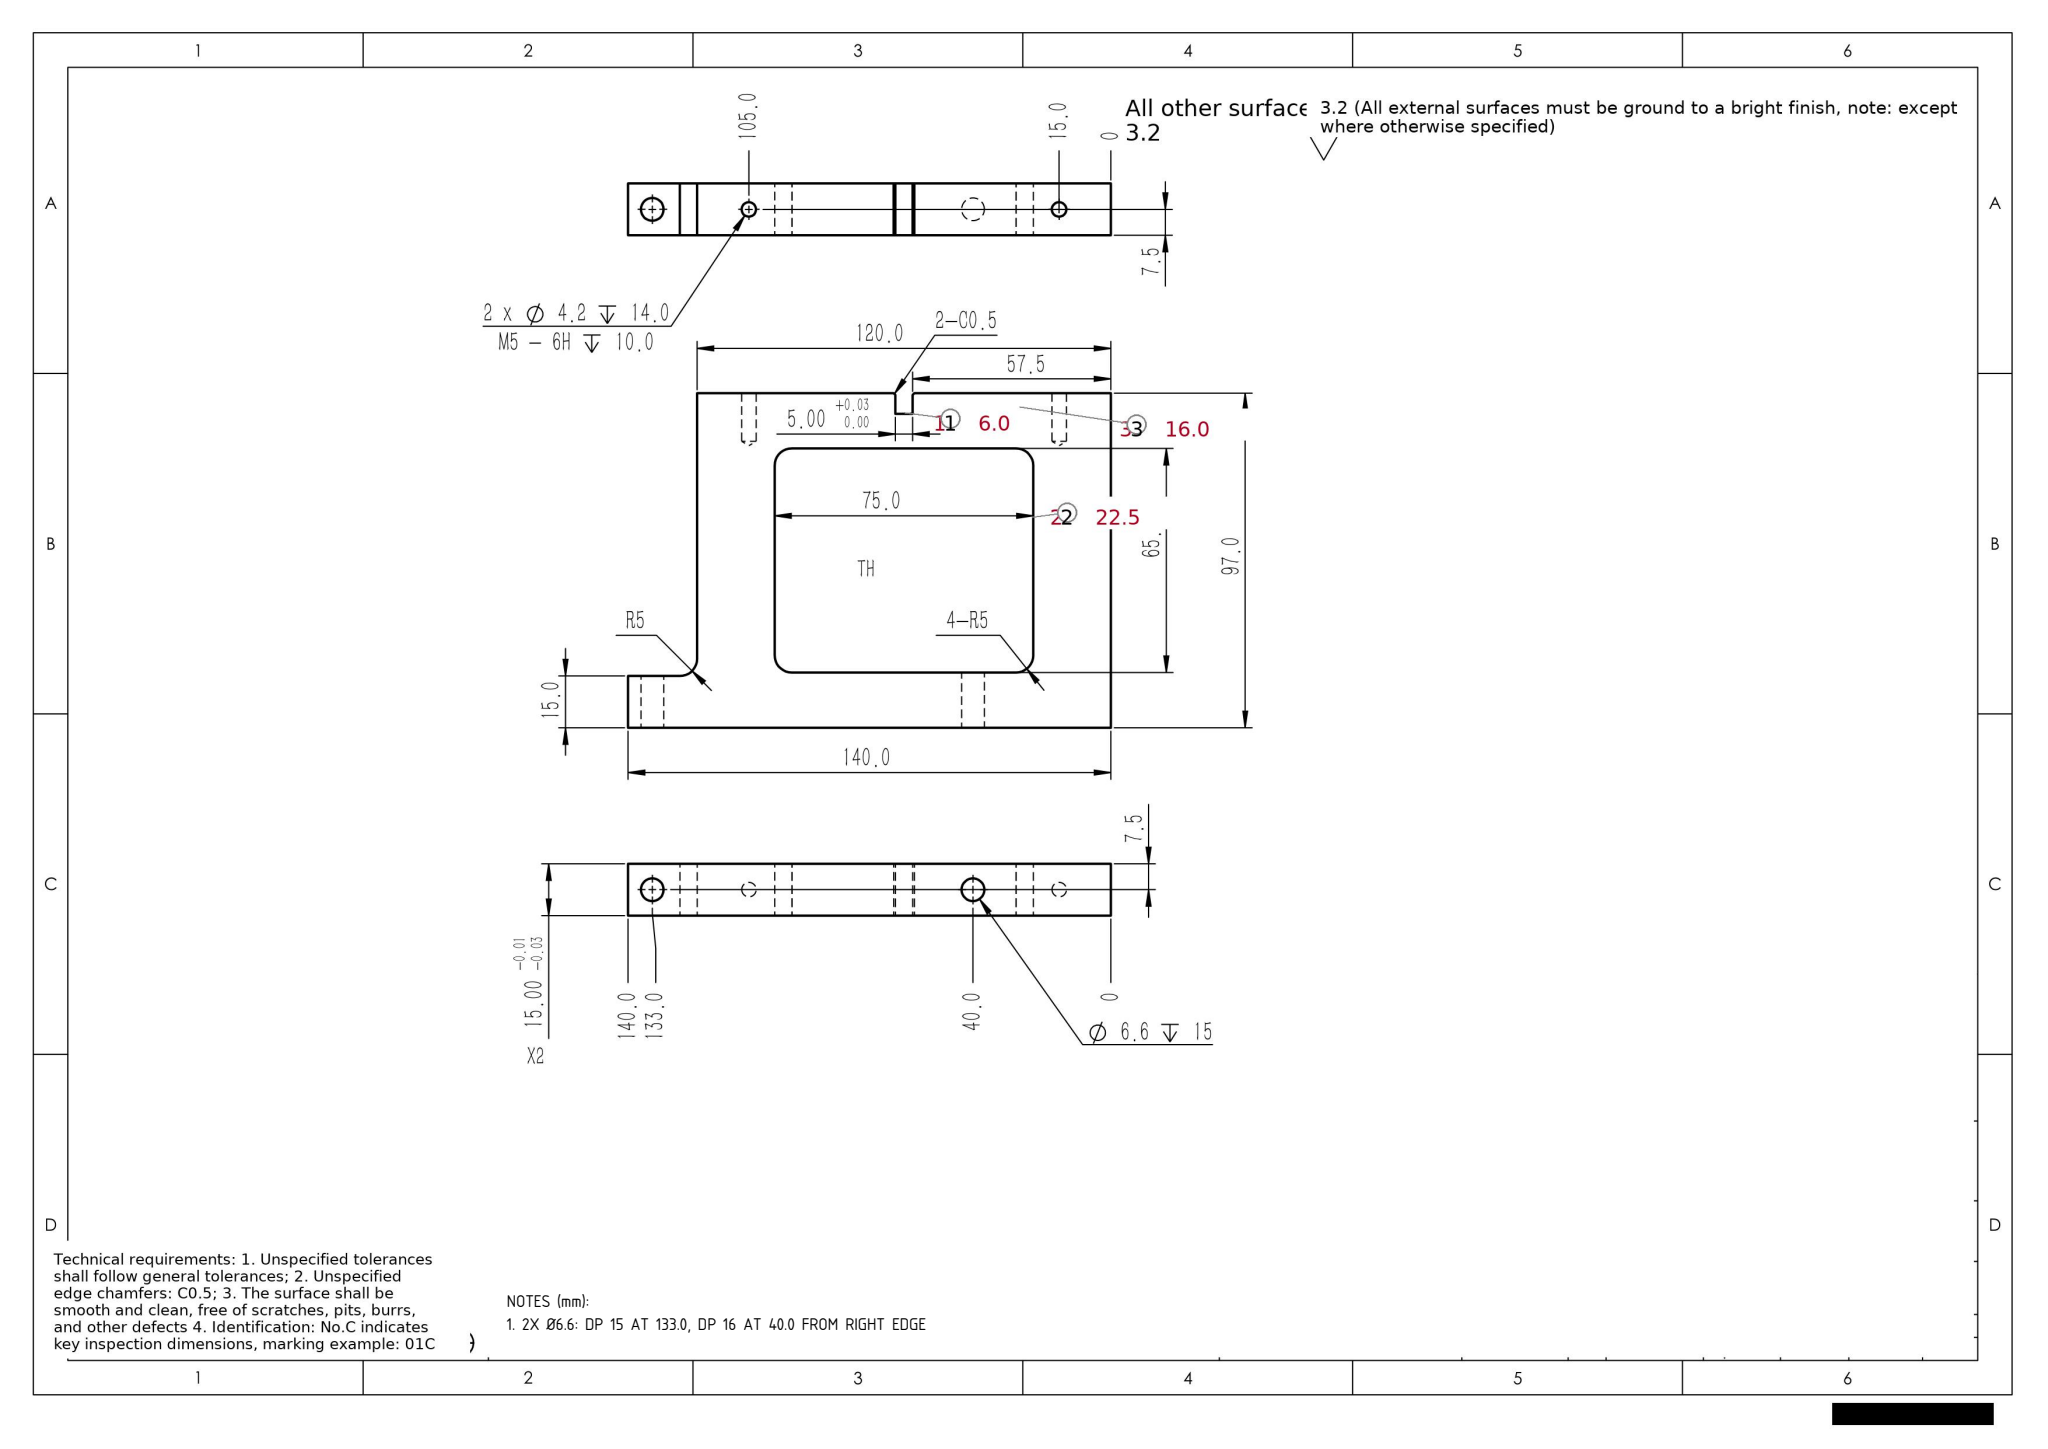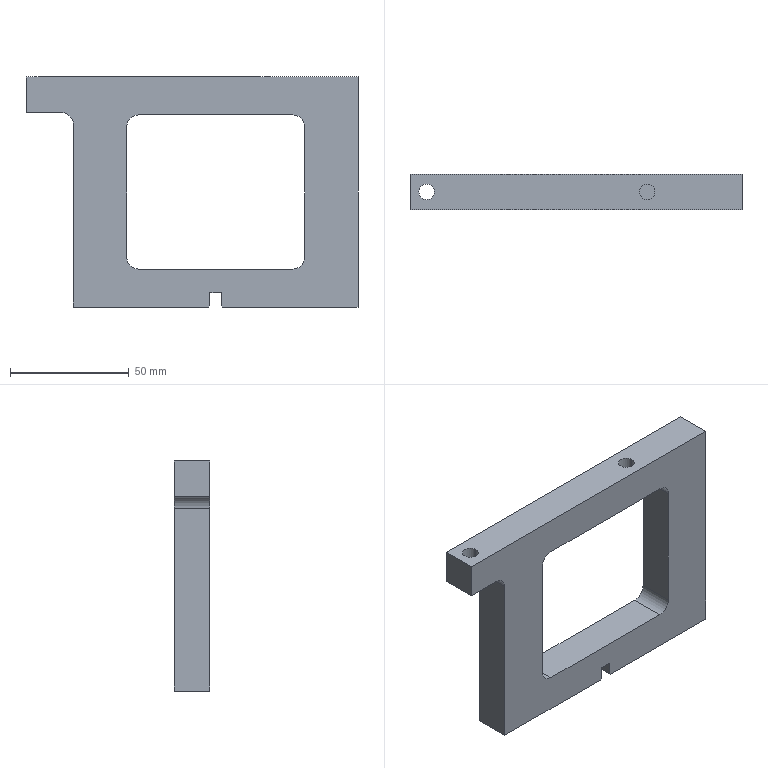Part | SolidWorks | mm | 1 solid | 35 faces | box 140 x 15 x 97 mm | volume 104463 mm3 | plane 18 | cylinder 13 | cone 4 | commonest cylinder face diameters 10 x5 4.2 x4 6.6 x4
Drawing notes:
2X Ø6.6: DP 15 AT 133.0, DP 16 AT 40.0 FROM RIGHT EDGE | from the solid: cylinders 6.6 dia, z axis: pos x=7.0 len 15 (=133 from x=140 edge) and pos x=100.0 len 16 (=40 from x=140 edge), both at y=7.5
build123d program:
from build123d import *

# Parameters (mm, degrees)
SKETCH1_W                 = 160
SKETCH1_H                 = 97
BOSS_EXTRUDE1_DEPTH       = 15
SKETCH2_W                 = 20
SKETCH2_H                 = 82
CUT_EXTRUDE1_DEPTH        = 95.748
FILLET1_R                 = 5
M6_CLEARANCE_HOLE_1_D     = 6.6
SKETCH5_W                 = 75
SKETCH5_H                 = 65
CUT_EXTRUDE2_DEPTH        = 95.748
FILLET2_R                 = 5
SKETCH6_W                 = 20
SKETCH6_H                 = 24
CUT_EXTRUDE3_DEPTH        = 95.748
M6_CLEARANCE_HOLE_2_D     = 6.6
M6_CLEARANCE_HOLE_2_DEPTH = 20
M6_CLEARANCE_HOLE_2_TIP   = 1.983
SKETCH10_W                = 5
SKETCH10_H                = 12
CUT_EXTRUDE4_DEPTH        = 95.748
CHAMFER1_SIZE             = 0.5
M5_TAPPED_HOLE1_D         = 4.2
M5_TAPPED_HOLE1_DEPTH     = 14
M5_TAPPED_HOLE1_TIP       = 1.262


with BuildPart() as part:
    # Sketch1 → Boss-Extrude1 (new body)
    with BuildSketch(Plane(origin=(0, 0, 0), x_dir=(1, 0, 0), z_dir=(0, 1, 0))):
        Rectangle(SKETCH1_W, SKETCH1_H)
    extrude(amount=BOSS_EXTRUDE1_DEPTH)

    # Sketch2 → Cut-Extrude1 (cut, through all)
    with BuildSketch(Plane(origin=(0, 15, 0), x_dir=(1, 0, 0), z_dir=(0, 1, 0))):
        with Locations((70, 7.5)):
            Rectangle(SKETCH2_W, SKETCH2_H)
        with Locations((-70, 7.5)):
            Rectangle(SKETCH2_W, SKETCH2_H)
    extrude(amount=-CUT_EXTRUDE1_DEPTH, mode=Mode.SUBTRACT)

    # Fillet1
    fillet1_edges = [part.edges().sort_by_distance(p)[0] for p in [
        (60, 7.5, 33.5),
        (-60, 7.5, 33.5),
    ]]
    fillet(fillet1_edges, radius=FILLET1_R)

    # M6 Clearance Hole 1 (through all)
    with Locations(Plane(origin=(0, 0, 33.5), x_dir=(-1, 0, 0), z_dir=(0, 0, -1))):
        with Locations((-73, 7.5), (73, 7.5)):
            Hole(M6_CLEARANCE_HOLE_1_D / 2)

    # Sketch5 → Cut-Extrude2 (cut, through all)
    with BuildSketch(Plane(origin=(0, 15, 0), x_dir=(1, 0, 0), z_dir=(0, 1, 0))):
        Rectangle(SKETCH5_W, SKETCH5_H)
    extrude(amount=-CUT_EXTRUDE2_DEPTH, mode=Mode.SUBTRACT)

    # Fillet2
    fillet2_edges = [part.edges().sort_by_distance(p)[0] for p in [
        (37.5, 7.5, -32.5),
        (37.5, 7.5, 32.5),
        (-37.5, 7.5, 32.5),
        (-37.5, 7.5, -32.5),
    ]]
    fillet(fillet2_edges, radius=FILLET2_R)

    # Sketch6 → Cut-Extrude3 (cut, through all)
    with BuildSketch(Plane(origin=(0, 15, 0), x_dir=(1, 0, 0), z_dir=(0, 1, 0))):
        with Locations((70, -36.5)):
            Rectangle(SKETCH6_W, SKETCH6_H)
    extrude(amount=-CUT_EXTRUDE3_DEPTH, mode=Mode.SUBTRACT)

    # M6 Clearance Hole 2
    with Locations(Plane.XY.offset(48.5)):
        with Locations((20, 7.5)):
            Hole(M6_CLEARANCE_HOLE_2_D / 2, depth=M6_CLEARANCE_HOLE_2_DEPTH)
            with Locations((0, 0, -(M6_CLEARANCE_HOLE_2_DEPTH + M6_CLEARANCE_HOLE_2_TIP / 2))):  # 118° drill point
                Cone(0, M6_CLEARANCE_HOLE_2_D / 2, M6_CLEARANCE_HOLE_2_TIP, mode=Mode.SUBTRACT)

    # Sketch10 → Cut-Extrude4 (cut, through all)
    with BuildSketch(Plane(origin=(0, 15, 0), x_dir=(1, 0, 0), z_dir=(0, 1, 0))):
        with Locations((0, 48.5)):
            Rectangle(SKETCH10_W, SKETCH10_H)
    extrude(amount=-CUT_EXTRUDE4_DEPTH, mode=Mode.SUBTRACT)

    # Chamfer1
    chamfer1_edges = [part.edges().sort_by_distance(p)[0] for p in [
        (2.5, 7.5, -48.5),
        (-2.5, 7.5, -48.5),
    ]]
    chamfer(chamfer1_edges, length=CHAMFER1_SIZE)

    # M5 Tapped Hole1
    with Locations(Plane(origin=(0, 0, -48.5), x_dir=(-1, 0, 0), z_dir=(0, 0, -1))):
        with Locations((-45, 7.5), (45, 7.5)):
            Hole(M5_TAPPED_HOLE1_D / 2, depth=M5_TAPPED_HOLE1_DEPTH)
            with Locations((0, 0, -(M5_TAPPED_HOLE1_DEPTH + M5_TAPPED_HOLE1_TIP / 2))):  # 118° drill point
                Cone(0, M5_TAPPED_HOLE1_D / 2, M5_TAPPED_HOLE1_TIP, mode=Mode.SUBTRACT)


solid = part.part